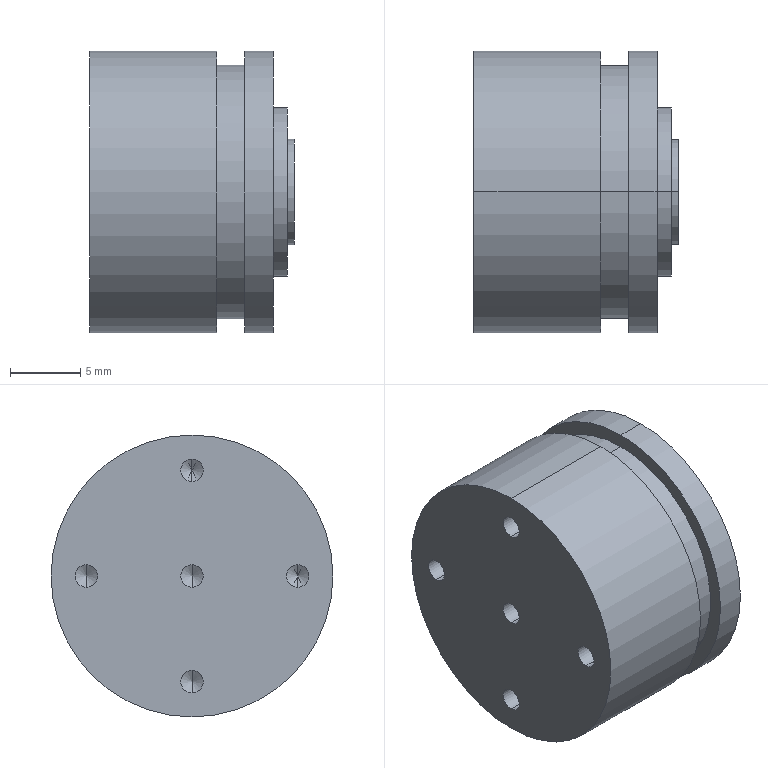Component | SolidWorks | WheelAssembly-1_PressureSensor-1 | 1 solid | 36 faces | box 14.5 x 20 x 20 mm | volume 4051 mm3 | cylinder 20 | cone 10 | plane 6 | commonest cylinder face diameters 1.6 x10 20 x4 7.5 x2 12 x2 18 x2
build123d program:
from build123d import *

# Parameters (mm, degrees)
SKETCH1_R             = 10
BOSS_EXTRUDE1_DEPTH   = 13
CUT_EXTRUDE1_START    = -4
SKETCH2_R             = 10
SKETCH2_R_2           = 9
CUT_EXTRUDE1_DEPTH    = 2
SKETCH3_R             = 6
BOSS_EXTRUDE2_DEPTH   = 1
SKETCH5_R             = 3.75
BOSS_EXTRUDE4_DEPTH   = 0.5
M2_TAPPED_HOLE1_D     = 1.6
M2_TAPPED_HOLE1_DEPTH = 4.7
M2_TAPPED_HOLE1_TIP   = 0.4807


with BuildPart() as part:
    # Sketch1 → Boss-Extrude1 (new body)
    with BuildSketch(Plane.XY):
        with Locations(Location((0, 0, 0), (0, 0, 180))):
            Circle(SKETCH1_R)
    extrude(amount=BOSS_EXTRUDE1_DEPTH)

    # Sketch2 → Cut-Extrude1 (cut)
    with BuildSketch(Plane.XY.offset(13).offset(CUT_EXTRUDE1_START)):
        with Locations(Location((0, 0, 0), (0, 0, 180))):
            Circle(SKETCH2_R)
        Circle(SKETCH2_R_2, mode=Mode.SUBTRACT)
    extrude(amount=CUT_EXTRUDE1_DEPTH, mode=Mode.SUBTRACT)

    # Sketch3 → Boss-Extrude2 (add)
    with BuildSketch(Plane.XY.offset(13)):
        Circle(SKETCH3_R)
    extrude(amount=BOSS_EXTRUDE2_DEPTH)

    # Sketch5 → Boss-Extrude4 (add)
    with BuildSketch(Plane.XY.offset(14)):
        Circle(SKETCH5_R)
    extrude(amount=BOSS_EXTRUDE4_DEPTH)

    # M2 Tapped Hole1
    with Locations(Plane(origin=(0, 0, 0), x_dir=(1, 0, 0), z_dir=(0, 0, -1))):
        with Locations((0, -7.5), (7.5, 0), (0, 7.5), (-7.5, 0), (0, 0)):
            Hole(M2_TAPPED_HOLE1_D / 2, depth=M2_TAPPED_HOLE1_DEPTH)
            with Locations((0, 0, -(M2_TAPPED_HOLE1_DEPTH + M2_TAPPED_HOLE1_TIP / 2))):  # 118° drill point
                Cone(0, M2_TAPPED_HOLE1_D / 2, M2_TAPPED_HOLE1_TIP, mode=Mode.SUBTRACT)


solid = part.part

# Placed as in the assembly
solid = solid.moved(Location((-376, -131.5, -542.97), (0, 90, 0)))
STEP:
#1=COLOUR_RGB('',0.7922,0.8196,0.9333);
#2=FILL_AREA_STYLE_COLOUR('',#1);
#3=FILL_AREA_STYLE('',(#2));
#4=SURFACE_STYLE_FILL_AREA(#3);
#5=SURFACE_SIDE_STYLE('',(#4));
#6=SURFACE_STYLE_USAGE(.BOTH.,#5);
#7=PRESENTATION_STYLE_ASSIGNMENT((#6));
#8=CARTESIAN_POINT('',(-14.618,-5.472,-21.345));
#9=VERTEX_POINT('',#8);
#10=CARTESIAN_POINT('',(-14.618,-5.472,-21.408));
#11=VERTEX_POINT('',#10);
#12=CARTESIAN_POINT('',(-14.618,-5.472,-21.377));
#13=DIRECTION('',(-1.,-0.,0.));
#14=DIRECTION('',(0.,0.,-1.));
#15=AXIS2_PLACEMENT_3D('',#12,#13,#14);
#16=CIRCLE('',#15,0.0315);
#17=EDGE_CURVE('',#9,#11,#16,.T.);
#18=ORIENTED_EDGE('',*,*,#17,.F.);
#19=CARTESIAN_POINT('',(-14.803,-5.472,-21.345));
#20=VERTEX_POINT('',#19);
#21=CARTESIAN_POINT('',(-14.803,-5.472,-21.345));
#22=DIRECTION('',(-1.,-0.,0.));
#23=VECTOR('',#22,39.37);
#24=LINE('',#21,#23);
#25=EDGE_CURVE('',#9,#20,#24,.T.);
#26=ORIENTED_EDGE('',*,*,#25,.T.);
#27=CARTESIAN_POINT('',(-14.803,-5.472,-21.408));
#28=VERTEX_POINT('',#27);
#29=CARTESIAN_POINT('',(-14.803,-5.472,-21.377));
#30=DIRECTION('',(-1.,-0.,0.));
#31=DIRECTION('',(0.,0.,-1.));
#32=AXIS2_PLACEMENT_3D('',#29,#30,#31);
#33=CIRCLE('',#32,0.0315);
#34=EDGE_CURVE('',#20,#28,#33,.T.);
#35=ORIENTED_EDGE('',*,*,#34,.T.);
#36=CARTESIAN_POINT('',(-14.803,-5.472,-21.408));
#37=DIRECTION('',(-1.,-0.,0.));
#38=VECTOR('',#37,39.37);
#39=LINE('',#36,#38);
#40=EDGE_CURVE('',#11,#28,#39,.T.);
#41=ORIENTED_EDGE('',*,*,#40,.F.);
#42=EDGE_LOOP('',(#18,#26,#35,#41));
#43=FACE_OUTER_BOUND('',#42,.T.);
#44=CARTESIAN_POINT('',(-14.803,-5.472,-21.377));
#45=DIRECTION('',(-1.,-0.,0.));
#46=DIRECTION('',(0.,0.,-1.));
#47=AXIS2_PLACEMENT_3D('',#44,#45,#46);
#48=CYLINDRICAL_SURFACE('',#47,0.0315);
#49=ADVANCED_FACE('',(#43),#48,.F.);
#50=CARTESIAN_POINT('',(-14.599,-5.472,-21.377));
#51=VERTEX_POINT('',#50);
#52=CARTESIAN_POINT('',(-14.618,-5.472,-21.408));
#53=DIRECTION('',(-0.515,-0.,-0.8572));
#54=VECTOR('',#53,39.37);
#55=LINE('',#52,#54);
#56=EDGE_CURVE('',#51,#11,#55,.T.);
#57=ORIENTED_EDGE('',*,*,#56,.F.);
#58=CARTESIAN_POINT('',(-14.618,-5.472,-21.345));
#59=DIRECTION('',(-0.515,0.,0.8572));
#60=VECTOR('',#59,39.37);
#61=LINE('',#58,#60);
#62=EDGE_CURVE('',#51,#9,#61,.T.);
#63=ORIENTED_EDGE('',*,*,#62,.T.);
#64=ORIENTED_EDGE('',*,*,#17,.T.);
#65=EDGE_LOOP('',(#57,#63,#64));
#66=FACE_OUTER_BOUND('',#65,.T.);
#67=CARTESIAN_POINT('',(-14.618,-5.472,-21.377));
#68=DIRECTION('',(-1.,-0.,0.));
#69=DIRECTION('',(0.,0.,-1.));
#70=AXIS2_PLACEMENT_3D('',#67,#68,#69);
#71=CONICAL_SURFACE('',#70,0.0315,1.03);
#72=ADVANCED_FACE('',(#66),#71,.F.);
#73=CARTESIAN_POINT('',(-14.618,-5.177,-21.05));
#74=VERTEX_POINT('',#73);
#75=CARTESIAN_POINT('',(-14.618,-5.177,-21.113));
#76=VERTEX_POINT('',#75);
#77=CARTESIAN_POINT('',(-14.618,-5.177,-21.081));
#78=DIRECTION('',(-1.,-0.,0.));
#79=DIRECTION('',(0.,0.,-1.));
#80=AXIS2_PLACEMENT_3D('',#77,#78,#79);
#81=CIRCLE('',#80,0.0315);
#82=EDGE_CURVE('',#74,#76,#81,.T.);
#83=ORIENTED_EDGE('',*,*,#82,.F.);
#84=CARTESIAN_POINT('',(-14.803,-5.177,-21.05));
#85=VERTEX_POINT('',#84);
#86=CARTESIAN_POINT('',(-14.803,-5.177,-21.05));
#87=DIRECTION('',(-1.,-0.,0.));
#88=VECTOR('',#87,39.37);
#89=LINE('',#86,#88);
#90=EDGE_CURVE('',#74,#85,#89,.T.);
#91=ORIENTED_EDGE('',*,*,#90,.T.);
#92=CARTESIAN_POINT('',(-14.803,-5.177,-21.113));
#93=VERTEX_POINT('',#92);
#94=CARTESIAN_POINT('',(-14.803,-5.177,-21.081));
#95=DIRECTION('',(-1.,-0.,0.));
#96=DIRECTION('',(0.,0.,-1.));
#97=AXIS2_PLACEMENT_3D('',#94,#95,#96);
#98=CIRCLE('',#97,0.0315);
#99=EDGE_CURVE('',#85,#93,#98,.T.);
#100=ORIENTED_EDGE('',*,*,#99,.T.);
#101=CARTESIAN_POINT('',(-14.803,-5.177,-21.113));
#102=DIRECTION('',(-1.,-0.,0.));
#103=VECTOR('',#102,39.37);
#104=LINE('',#101,#103);
#105=EDGE_CURVE('',#76,#93,#104,.T.);
#106=ORIENTED_EDGE('',*,*,#105,.F.);
#107=EDGE_LOOP('',(#83,#91,#100,#106));
#108=FACE_OUTER_BOUND('',#107,.T.);
#109=CARTESIAN_POINT('',(-14.803,-5.177,-21.081));
#110=DIRECTION('',(-1.,-0.,0.));
#111=DIRECTION('',(0.,0.,-1.));
#112=AXIS2_PLACEMENT_3D('',#109,#110,#111);
#113=CYLINDRICAL_SURFACE('',#112,0.0315);
#114=ADVANCED_FACE('',(#108),#113,.F.);
#115=CARTESIAN_POINT('',(-14.599,-5.177,-21.081));
#116=VERTEX_POINT('',#115);
#117=CARTESIAN_POINT('',(-14.618,-5.177,-21.113));
#118=DIRECTION('',(-0.515,-0.,-0.8572));
#119=VECTOR('',#118,39.37);
#120=LINE('',#117,#119);
#121=EDGE_CURVE('',#116,#76,#120,.T.);
#122=ORIENTED_EDGE('',*,*,#121,.F.);
#123=CARTESIAN_POINT('',(-14.618,-5.177,-21.05));
#124=DIRECTION('',(-0.515,0.,0.8572));
#125=VECTOR('',#124,39.37);
#126=LINE('',#123,#125);
#127=EDGE_CURVE('',#116,#74,#126,.T.);
#128=ORIENTED_EDGE('',*,*,#127,.T.);
#129=ORIENTED_EDGE('',*,*,#82,.T.);
#130=EDGE_LOOP('',(#122,#128,#129));
#131=FACE_OUTER_BOUND('',#130,.T.);
#132=CARTESIAN_POINT('',(-14.618,-5.177,-21.081));
#133=DIRECTION('',(-1.,-0.,0.));
#134=DIRECTION('',(0.,0.,-1.));
#135=AXIS2_PLACEMENT_3D('',#132,#133,#134);
#136=CONICAL_SURFACE('',#135,0.0315,1.03);
#137=ADVANCED_FACE('',(#131),#136,.F.);
#138=CARTESIAN_POINT('',(-14.618,-4.882,-21.345));
#139=VERTEX_POINT('',#138);
#140=CARTESIAN_POINT('',(-14.618,-4.882,-21.408));
#141=VERTEX_POINT('',#140);
#142=CARTESIAN_POINT('',(-14.618,-4.882,-21.377));
#143=DIRECTION('',(-1.,-0.,0.));
#144=DIRECTION('',(0.,0.,-1.));
#145=AXIS2_PLACEMENT_3D('',#142,#143,#144);
#146=CIRCLE('',#145,0.0315);
#147=EDGE_CURVE('',#139,#141,#146,.T.);
#148=ORIENTED_EDGE('',*,*,#147,.F.);
#149=CARTESIAN_POINT('',(-14.803,-4.882,-21.345));
#150=VERTEX_POINT('',#149);
#151=CARTESIAN_POINT('',(-14.803,-4.882,-21.345));
#152=DIRECTION('',(-1.,-0.,0.));
#153=VECTOR('',#152,39.37);
#154=LINE('',#151,#153);
#155=EDGE_CURVE('',#139,#150,#154,.T.);
#156=ORIENTED_EDGE('',*,*,#155,.T.);
#157=CARTESIAN_POINT('',(-14.803,-4.882,-21.408));
#158=VERTEX_POINT('',#157);
#159=CARTESIAN_POINT('',(-14.803,-4.882,-21.377));
#160=DIRECTION('',(-1.,-0.,0.));
#161=DIRECTION('',(0.,0.,-1.));
#162=AXIS2_PLACEMENT_3D('',#159,#160,#161);
#163=CIRCLE('',#162,0.0315);
#164=EDGE_CURVE('',#150,#158,#163,.T.);
#165=ORIENTED_EDGE('',*,*,#164,.T.);
#166=CARTESIAN_POINT('',(-14.803,-4.882,-21.408));
#167=DIRECTION('',(-1.,-0.,0.));
#168=VECTOR('',#167,39.37);
#169=LINE('',#166,#168);
#170=EDGE_CURVE('',#141,#158,#169,.T.);
#171=ORIENTED_EDGE('',*,*,#170,.F.);
#172=EDGE_LOOP('',(#148,#156,#165,#171));
#173=FACE_OUTER_BOUND('',#172,.T.);
#174=CARTESIAN_POINT('',(-14.803,-4.882,-21.377));
#175=DIRECTION('',(-1.,-0.,0.));
#176=DIRECTION('',(0.,0.,-1.));
#177=AXIS2_PLACEMENT_3D('',#174,#175,#176);
#178=CYLINDRICAL_SURFACE('',#177,0.0315);
#179=ADVANCED_FACE('',(#173),#178,.F.);
#180=CARTESIAN_POINT('',(-14.599,-4.882,-21.377));
#181=VERTEX_POINT('',#180);
#182=CARTESIAN_POINT('',(-14.618,-4.882,-21.408));
#183=DIRECTION('',(-0.515,-0.,-0.8572));
#184=VECTOR('',#183,39.37);
#185=LINE('',#182,#184);
#186=EDGE_CURVE('',#181,#141,#185,.T.);
#187=ORIENTED_EDGE('',*,*,#186,.F.);
#188=CARTESIAN_POINT('',(-14.618,-4.882,-21.345));
#189=DIRECTION('',(-0.515,0.,0.8572));
#190=VECTOR('',#189,39.37);
#191=LINE('',#188,#190);
#192=EDGE_CURVE('',#181,#139,#191,.T.);
#193=ORIENTED_EDGE('',*,*,#192,.T.);
#194=ORIENTED_EDGE('',*,*,#147,.T.);
#195=EDGE_LOOP('',(#187,#193,#194));
#196=FACE_OUTER_BOUND('',#195,.T.);
#197=CARTESIAN_POINT('',(-14.618,-4.882,-21.377));
#198=DIRECTION('',(-1.,-0.,0.));
#199=DIRECTION('',(0.,0.,-1.));
#200=AXIS2_PLACEMENT_3D('',#197,#198,#199);
#201=CONICAL_SURFACE('',#200,0.0315,1.03);
#202=ADVANCED_FACE('',(#196),#201,.F.);
#203=CARTESIAN_POINT('',(-14.618,-5.177,-21.641));
#204=VERTEX_POINT('',#203);
#205=CARTESIAN_POINT('',(-14.618,-5.177,-21.704));
#206=VERTEX_POINT('',#205);
#207=CARTESIAN_POINT('',(-14.618,-5.177,-21.672));
#208=DIRECTION('',(-1.,-0.,0.));
#209=DIRECTION('',(0.,0.,-1.));
#210=AXIS2_PLACEMENT_3D('',#207,#208,#209);
#211=CIRCLE('',#210,0.0315);
#212=EDGE_CURVE('',#204,#206,#211,.T.);
#213=ORIENTED_EDGE('',*,*,#212,.F.);
#214=CARTESIAN_POINT('',(-14.803,-5.177,-21.641));
#215=VERTEX_POINT('',#214);
#216=CARTESIAN_POINT('',(-14.803,-5.177,-21.641));
#217=DIRECTION('',(-1.,-0.,0.));
#218=VECTOR('',#217,39.37);
#219=LINE('',#216,#218);
#220=EDGE_CURVE('',#204,#215,#219,.T.);
#221=ORIENTED_EDGE('',*,*,#220,.T.);
#222=CARTESIAN_POINT('',(-14.803,-5.177,-21.704));
#223=VERTEX_POINT('',#222);
#224=CARTESIAN_POINT('',(-14.803,-5.177,-21.672));
#225=DIRECTION('',(-1.,-0.,0.));
#226=DIRECTION('',(0.,0.,-1.));
#227=AXIS2_PLACEMENT_3D('',#224,#225,#226);
#228=CIRCLE('',#227,0.0315);
#229=EDGE_CURVE('',#215,#223,#228,.T.);
#230=ORIENTED_EDGE('',*,*,#229,.T.);
#231=CARTESIAN_POINT('',(-14.803,-5.177,-21.704));
#232=DIRECTION('',(-1.,-0.,0.));
#233=VECTOR('',#232,39.37);
#234=LINE('',#231,#233);
#235=EDGE_CURVE('',#206,#223,#234,.T.);
#236=ORIENTED_EDGE('',*,*,#235,.F.);
#237=EDGE_LOOP('',(#213,#221,#230,#236));
#238=FACE_OUTER_BOUND('',#237,.T.);
#239=CARTESIAN_POINT('',(-14.803,-5.177,-21.672));
#240=DIRECTION('',(-1.,-0.,0.));
#241=DIRECTION('',(0.,0.,-1.));
#242=AXIS2_PLACEMENT_3D('',#239,#240,#241);
#243=CYLINDRICAL_SURFACE('',#242,0.0315);
#244=ADVANCED_FACE('',(#238),#243,.F.);
#245=CARTESIAN_POINT('',(-14.599,-5.177,-21.672));
#246=VERTEX_POINT('',#245);
#247=CARTESIAN_POINT('',(-14.618,-5.177,-21.704));
#248=DIRECTION('',(-0.515,-0.,-0.8572));
#249=VECTOR('',#248,39.37);
#250=LINE('',#247,#249);
#251=EDGE_CURVE('',#246,#206,#250,.T.);
#252=ORIENTED_EDGE('',*,*,#251,.F.);
#253=CARTESIAN_POINT('',(-14.618,-5.177,-21.641));
#254=DIRECTION('',(-0.515,0.,0.8572));
#255=VECTOR('',#254,39.37);
#256=LINE('',#253,#255);
#257=EDGE_CURVE('',#246,#204,#256,.T.);
#258=ORIENTED_EDGE('',*,*,#257,.T.);
#259=ORIENTED_EDGE('',*,*,#212,.T.);
#260=EDGE_LOOP('',(#252,#258,#259));
#261=FACE_OUTER_BOUND('',#260,.T.);
#262=CARTESIAN_POINT('',(-14.618,-5.177,-21.672));
#263=DIRECTION('',(-1.,-0.,0.));
#264=DIRECTION('',(0.,0.,-1.));
#265=AXIS2_PLACEMENT_3D('',#262,#263,#264);
#266=CONICAL_SURFACE('',#265,0.0315,1.03);
#267=ADVANCED_FACE('',(#261),#266,.F.);
#268=CARTESIAN_POINT('',(-14.618,-5.177,-21.345));
#269=VERTEX_POINT('',#268);
#270=CARTESIAN_POINT('',(-14.618,-5.177,-21.408));
#271=VERTEX_POINT('',#270);
#272=CARTESIAN_POINT('',(-14.618,-5.177,-21.377));
#273=DIRECTION('',(-1.,-0.,0.));
#274=DIRECTION('',(0.,0.,-1.));
#275=AXIS2_PLACEMENT_3D('',#272,#273,#274);
#276=CIRCLE('',#275,0.0315);
#277=EDGE_CURVE('',#269,#271,#276,.T.);
#278=ORIENTED_EDGE('',*,*,#277,.F.);
#279=CARTESIAN_POINT('',(-14.803,-5.177,-21.345));
#280=VERTEX_POINT('',#279);
#281=CARTESIAN_POINT('',(-14.803,-5.177,-21.345));
#282=DIRECTION('',(-1.,-0.,0.));
#283=VECTOR('',#282,39.37);
#284=LINE('',#281,#283);
#285=EDGE_CURVE('',#269,#280,#284,.T.);
#286=ORIENTED_EDGE('',*,*,#285,.T.);
#287=CARTESIAN_POINT('',(-14.803,-5.177,-21.408));
#288=VERTEX_POINT('',#287);
#289=CARTESIAN_POINT('',(-14.803,-5.177,-21.377));
#290=DIRECTION('',(-1.,-0.,0.));
#291=DIRECTION('',(0.,0.,-1.));
#292=AXIS2_PLACEMENT_3D('',#289,#290,#291);
#293=CIRCLE('',#292,0.0315);
#294=EDGE_CURVE('',#280,#288,#293,.T.);
#295=ORIENTED_EDGE('',*,*,#294,.T.);
#296=CARTESIAN_POINT('',(-14.803,-5.177,-21.408));
#297=DIRECTION('',(-1.,-0.,0.));
#298=VECTOR('',#297,39.37);
#299=LINE('',#296,#298);
#300=EDGE_CURVE('',#271,#288,#299,.T.);
#301=ORIENTED_EDGE('',*,*,#300,.F.);
#302=EDGE_LOOP('',(#278,#286,#295,#301));
#303=FACE_OUTER_BOUND('',#302,.T.);
#304=CARTESIAN_POINT('',(-14.803,-5.177,-21.377));
#305=DIRECTION('',(-1.,-0.,0.));
#306=DIRECTION('',(0.,0.,-1.));
#307=AXIS2_PLACEMENT_3D('',#304,#305,#306);
#308=CYLINDRICAL_SURFACE('',#307,0.0315);
#309=ADVANCED_FACE('',(#303),#308,.F.);
#310=CARTESIAN_POINT('',(-14.599,-5.177,-21.377));
#311=VERTEX_POINT('',#310);
#312=CARTESIAN_POINT('',(-14.618,-5.177,-21.408));
#313=DIRECTION('',(-0.515,-0.,-0.8572));
#314=VECTOR('',#313,39.37);
#315=LINE('',#312,#314);
#316=EDGE_CURVE('',#311,#271,#315,.T.);
#317=ORIENTED_EDGE('',*,*,#316,.F.);
#318=CARTESIAN_POINT('',(-14.618,-5.177,-21.345));
#319=DIRECTION('',(-0.515,0.,0.8572));
#320=VECTOR('',#319,39.37);
#321=LINE('',#318,#320);
#322=EDGE_CURVE('',#311,#269,#321,.T.);
#323=ORIENTED_EDGE('',*,*,#322,.T.);
#324=ORIENTED_EDGE('',*,*,#277,.T.);
#325=EDGE_LOOP('',(#317,#323,#324));
#326=FACE_OUTER_BOUND('',#325,.T.);
#327=CARTESIAN_POINT('',(-14.618,-5.177,-21.377));
#328=DIRECTION('',(-1.,-0.,0.));
#329=DIRECTION('',(0.,0.,-1.));
#330=AXIS2_PLACEMENT_3D('',#327,#328,#329);
#331=CONICAL_SURFACE('',#330,0.0315,1.03);
#332=ADVANCED_FACE('',(#326),#331,.F.);
#333=CARTESIAN_POINT('',(-14.232,-5.177,-21.229));
#334=VERTEX_POINT('',#333);
#335=CARTESIAN_POINT('',(-14.232,-5.177,-21.524));
#336=VERTEX_POINT('',#335);
#337=CARTESIAN_POINT('',(-14.232,-5.177,-21.377));
#338=DIRECTION('',(1.,0.,-0.));
#339=DIRECTION('',(0.,0.,1.));
#340=AXIS2_PLACEMENT_3D('',#337,#338,#339);
#341=CIRCLE('',#340,0.1476);
#342=EDGE_CURVE('',#334,#336,#341,.T.);
#343=ORIENTED_EDGE('',*,*,#342,.F.);
#344=CARTESIAN_POINT('',(-14.252,-5.177,-21.229));
#345=VERTEX_POINT('',#344);
#346=CARTESIAN_POINT('',(-14.232,-5.177,-21.229));
#347=DIRECTION('',(-1.,-0.,0.));
#348=VECTOR('',#347,39.37);
#349=LINE('',#346,#348);
#350=EDGE_CURVE('',#334,#345,#349,.T.);
#351=ORIENTED_EDGE('',*,*,#350,.T.);
#352=CARTESIAN_POINT('',(-14.252,-5.177,-21.524));
#353=VERTEX_POINT('',#352);
#354=CARTESIAN_POINT('',(-14.252,-5.177,-21.377));
#355=DIRECTION('',(1.,0.,-0.));
#356=DIRECTION('',(0.,0.,1.));
#357=AXIS2_PLACEMENT_3D('',#354,#355,#356);
#358=CIRCLE('',#357,0.1476);
#359=EDGE_CURVE('',#345,#353,#358,.T.);
#360=ORIENTED_EDGE('',*,*,#359,.T.);
#361=CARTESIAN_POINT('',(-14.232,-5.177,-21.524));
#362=DIRECTION('',(-1.,-0.,0.));
#363=VECTOR('',#362,39.37);
#364=LINE('',#361,#363);
#365=EDGE_CURVE('',#336,#353,#364,.T.);
#366=ORIENTED_EDGE('',*,*,#365,.F.);
#367=EDGE_LOOP('',(#343,#351,#360,#366));
#368=FACE_OUTER_BOUND('',#367,.T.);
#369=CARTESIAN_POINT('',(-14.232,-5.177,-21.377));
#370=DIRECTION('',(-1.,-0.,0.));
#371=DIRECTION('',(0.,-0.,-1.));
#372=AXIS2_PLACEMENT_3D('',#369,#370,#371);
#373=CYLINDRICAL_SURFACE('',#372,0.1476);
#374=ADVANCED_FACE('',(#368),#373,.T.);
#375=CARTESIAN_POINT('',(-14.252,-5.177,-21.141));
#376=VERTEX_POINT('',#375);
#377=CARTESIAN_POINT('',(-14.252,-5.177,-21.613));
#378=VERTEX_POINT('',#377);
#379=CARTESIAN_POINT('',(-14.252,-5.177,-21.377));
#380=DIRECTION('',(1.,0.,-0.));
#381=DIRECTION('',(0.,0.,1.));
#382=AXIS2_PLACEMENT_3D('',#379,#380,#381);
#383=CIRCLE('',#382,0.2362);
#384=EDGE_CURVE('',#376,#378,#383,.T.);
#385=ORIENTED_EDGE('',*,*,#384,.F.);
#386=CARTESIAN_POINT('',(-14.291,-5.177,-21.141));
#387=VERTEX_POINT('',#386);
#388=CARTESIAN_POINT('',(-14.252,-5.177,-21.141));
#389=DIRECTION('',(-1.,-0.,0.));
#390=VECTOR('',#389,39.37);
#391=LINE('',#388,#390);
#392=EDGE_CURVE('',#376,#387,#391,.T.);
#393=ORIENTED_EDGE('',*,*,#392,.T.);
#394=CARTESIAN_POINT('',(-14.291,-5.177,-21.613));
#395=VERTEX_POINT('',#394);
#396=CARTESIAN_POINT('',(-14.291,-5.177,-21.377));
#397=DIRECTION('',(1.,0.,-0.));
#398=DIRECTION('',(0.,0.,1.));
#399=AXIS2_PLACEMENT_3D('',#396,#397,#398);
#400=CIRCLE('',#399,0.2362);
#401=EDGE_CURVE('',#387,#395,#400,.T.);
#402=ORIENTED_EDGE('',*,*,#401,.T.);
#403=CARTESIAN_POINT('',(-14.252,-5.177,-21.613));
#404=DIRECTION('',(-1.,-0.,0.));
#405=VECTOR('',#404,39.37);
#406=LINE('',#403,#405);
#407=EDGE_CURVE('',#378,#395,#406,.T.);
#408=ORIENTED_EDGE('',*,*,#407,.F.);
#409=EDGE_LOOP('',(#385,#393,#402,#408));
#410=FACE_OUTER_BOUND('',#409,.T.);
#411=CARTESIAN_POINT('',(-14.252,-5.177,-21.377));
#412=DIRECTION('',(-1.,-0.,0.));
#413=DIRECTION('',(0.,-0.,-1.));
#414=AXIS2_PLACEMENT_3D('',#411,#412,#413);
#415=CYLINDRICAL_SURFACE('',#414,0.2362);
#416=ADVANCED_FACE('',(#410),#415,.T.);
#417=CARTESIAN_POINT('',(-14.291,-5.177,-20.983));
#418=VERTEX_POINT('',#417);
#419=CARTESIAN_POINT('',(-14.291,-5.177,-21.77));
#420=VERTEX_POINT('',#419);
#421=CARTESIAN_POINT('',(-14.291,-5.177,-21.377));
#422=DIRECTION('',(1.,0.,-0.));
#423=DIRECTION('',(0.,0.,1.));
#424=AXIS2_PLACEMENT_3D('',#421,#422,#423);
#425=CIRCLE('',#424,0.3937);
#426=EDGE_CURVE('',#418,#420,#425,.T.);
#427=ORIENTED_EDGE('',*,*,#426,.F.);
#428=CARTESIAN_POINT('',(-14.37,-5.177,-20.983));
#429=VERTEX_POINT('',#428);
#430=CARTESIAN_POINT('',(-14.291,-5.177,-20.983));
#431=DIRECTION('',(-1.,-0.,0.));
#432=VECTOR('',#431,39.37);
#433=LINE('',#430,#432);
#434=EDGE_CURVE('',#418,#429,#433,.T.);
#435=ORIENTED_EDGE('',*,*,#434,.T.);
#436=CARTESIAN_POINT('',(-14.37,-5.177,-21.77));
#437=VERTEX_POINT('',#436);
#438=CARTESIAN_POINT('',(-14.37,-5.177,-21.377));
#439=DIRECTION('',(1.,0.,-0.));
#440=DIRECTION('',(0.,0.,1.));
#441=AXIS2_PLACEMENT_3D('',#438,#439,#440);
#442=CIRCLE('',#441,0.3937);
#443=EDGE_CURVE('',#429,#437,#442,.T.);
#444=ORIENTED_EDGE('',*,*,#443,.T.);
#445=CARTESIAN_POINT('',(-14.291,-5.177,-21.77));
#446=DIRECTION('',(-1.,-0.,0.));
#447=VECTOR('',#446,39.37);
#448=LINE('',#445,#447);
#449=EDGE_CURVE('',#420,#437,#448,.T.);
#450=ORIENTED_EDGE('',*,*,#449,.F.);
#451=EDGE_LOOP('',(#427,#435,#444,#450));
#452=FACE_OUTER_BOUND('',#451,.T.);
#453=CARTESIAN_POINT('',(-14.291,-5.177,-21.377));
#454=DIRECTION('',(-1.,-0.,0.));
#455=DIRECTION('',(0.,-0.,-1.));
#456=AXIS2_PLACEMENT_3D('',#453,#454,#455);
#457=CYLINDRICAL_SURFACE('',#456,0.3937);
#458=ADVANCED_FACE('',(#452),#457,.T.);
#459=CARTESIAN_POINT('',(-14.449,-5.177,-21.022));
#460=VERTEX_POINT('',#459);
#461=CARTESIAN_POINT('',(-14.449,-5.177,-21.731));
#462=VERTEX_POINT('',#461);
#463=CARTESIAN_POINT('',(-14.449,-5.177,-21.377));
#464=DIRECTION('',(1.,0.,-0.));
#465=DIRECTION('',(0.,0.,1.));
#466=AXIS2_PLACEMENT_3D('',#463,#464,#465);
#467=CIRCLE('',#466,0.3543);
#468=EDGE_CURVE('',#460,#462,#467,.T.);
#469=ORIENTED_EDGE('',*,*,#468,.T.);
#470=CARTESIAN_POINT('',(-14.37,-5.177,-21.731));
#471=VERTEX_POINT('',#470);
#472=CARTESIAN_POINT('',(-14.449,-5.177,-21.731));
#473=DIRECTION('',(1.,0.,-0.));
#474=VECTOR('',#473,39.37);
#475=LINE('',#472,#474);
#476=EDGE_CURVE('',#462,#471,#475,.T.);
#477=ORIENTED_EDGE('',*,*,#476,.T.);
#478=CARTESIAN_POINT('',(-14.37,-5.177,-21.022));
#479=VERTEX_POINT('',#478);
#480=CARTESIAN_POINT('',(-14.37,-5.177,-21.377));
#481=DIRECTION('',(1.,0.,-0.));
#482=DIRECTION('',(0.,0.,1.));
#483=AXIS2_PLACEMENT_3D('',#480,#481,#482);
#484=CIRCLE('',#483,0.3543);
#485=EDGE_CURVE('',#479,#471,#484,.T.);
#486=ORIENTED_EDGE('',*,*,#485,.F.);
#487=CARTESIAN_POINT('',(-14.449,-5.177,-21.022));
#488=DIRECTION('',(1.,0.,-0.));
#489=VECTOR('',#488,39.37);
#490=LINE('',#487,#489);
#491=EDGE_CURVE('',#460,#479,#490,.T.);
#492=ORIENTED_EDGE('',*,*,#491,.F.);
#493=EDGE_LOOP('',(#469,#477,#486,#492));
#494=FACE_OUTER_BOUND('',#493,.T.);
#495=CARTESIAN_POINT('',(-14.449,-5.177,-21.377));
#496=DIRECTION('',(1.,0.,-0.));
#497=DIRECTION('',(0.,0.,1.));
#498=AXIS2_PLACEMENT_3D('',#495,#496,#497);
#499=CYLINDRICAL_SURFACE('',#498,0.3543);
#500=ADVANCED_FACE('',(#494),#499,.T.);
#501=CARTESIAN_POINT('',(-14.449,-5.177,-20.983));
#502=VERTEX_POINT('',#501);
#503=CARTESIAN_POINT('',(-14.449,-5.177,-21.77));
#504=VERTEX_POINT('',#503);
#505=CARTESIAN_POINT('',(-14.449,-5.177,-21.377));
#506=DIRECTION('',(1.,0.,-0.));
#507=DIRECTION('',(0.,0.,1.));
#508=AXIS2_PLACEMENT_3D('',#505,#506,#507);
#509=CIRCLE('',#508,0.3937);
#510=EDGE_CURVE('',#502,#504,#509,.T.);
#511=ORIENTED_EDGE('',*,*,#510,.F.);
#512=CARTESIAN_POINT('',(-14.803,-5.177,-20.983));
#513=VERTEX_POINT('',#512);
#514=CARTESIAN_POINT('',(-14.291,-5.177,-20.983));
#515=DIRECTION('',(-1.,-0.,0.));
#516=VECTOR('',#515,39.37);
#517=LINE('',#514,#516);
#518=EDGE_CURVE('',#502,#513,#517,.T.);
#519=ORIENTED_EDGE('',*,*,#518,.T.);
#520=CARTESIAN_POINT('',(-14.803,-5.177,-21.77));
#521=VERTEX_POINT('',#520);
#522=CARTESIAN_POINT('',(-14.803,-5.177,-21.377));
#523=DIRECTION('',(1.,0.,-0.));
#524=DIRECTION('',(0.,0.,1.));
#525=AXIS2_PLACEMENT_3D('',#522,#523,#524);
#526=CIRCLE('',#525,0.3937);
#527=EDGE_CURVE('',#513,#521,#526,.T.);
#528=ORIENTED_EDGE('',*,*,#527,.T.);
#529=CARTESIAN_POINT('',(-14.291,-5.177,-21.77));
#530=DIRECTION('',(-1.,-0.,0.));
#531=VECTOR('',#530,39.37);
#532=LINE('',#529,#531);
#533=EDGE_CURVE('',#504,#521,#532,.T.);
#534=ORIENTED_EDGE('',*,*,#533,.F.);
#535=EDGE_LOOP('',(#511,#519,#528,#534));
#536=FACE_OUTER_BOUND('',#535,.T.);
#537=CARTESIAN_POINT('',(-14.291,-5.177,-21.377));
#538=DIRECTION('',(-1.,-0.,0.));
#539=DIRECTION('',(0.,-0.,-1.));
#540=AXIS2_PLACEMENT_3D('',#537,#538,#539);
#541=CYLINDRICAL_SURFACE('',#540,0.3937);
#542=ADVANCED_FACE('',(#536),#541,.T.);
#543=CARTESIAN_POINT('',(-14.803,-5.472,-21.377));
#544=DIRECTION('',(-1.,-0.,0.));
#545=DIRECTION('',(0.,0.,-1.));
#546=AXIS2_PLACEMENT_3D('',#543,#544,#545);
#547=CIRCLE('',#546,0.0315);
#548=EDGE_CURVE('',#28,#20,#547,.T.);
#549=ORIENTED_EDGE('',*,*,#548,.F.);
#550=ORIENTED_EDGE('',*,*,#34,.F.);
#551=EDGE_LOOP('',(#549,#550));
#552=FACE_BOUND('',#551,.T.);
#553=CARTESIAN_POINT('',(-14.803,-5.177,-21.672));
#554=DIRECTION('',(-1.,-0.,0.));
#555=DIRECTION('',(0.,0.,-1.));
#556=AXIS2_PLACEMENT_3D('',#553,#554,#555);
#557=CIRCLE('',#556,0.0315);
#558=EDGE_CURVE('',#223,#215,#557,.T.);
#559=ORIENTED_EDGE('',*,*,#558,.F.);
#560=ORIENTED_EDGE('',*,*,#229,.F.);
#561=EDGE_LOOP('',(#559,#560));
#562=FACE_BOUND('',#561,.T.);
#563=CARTESIAN_POINT('',(-14.803,-5.177,-21.377));
#564=DIRECTION('',(-1.,-0.,0.));
#565=DIRECTION('',(0.,0.,-1.));
#566=AXIS2_PLACEMENT_3D('',#563,#564,#565);
#567=CIRCLE('',#566,0.0315);
#568=EDGE_CURVE('',#288,#280,#567,.T.);
#569=ORIENTED_EDGE('',*,*,#568,.F.);
#570=ORIENTED_EDGE('',*,*,#294,.F.);
#571=EDGE_LOOP('',(#569,#570));
#572=FACE_BOUND('',#571,.T.);
#573=CARTESIAN_POINT('',(-14.803,-5.177,-21.377));
#574=DIRECTION('',(1.,0.,-0.));
#575=DIRECTION('',(0.,0.,1.));
#576=AXIS2_PLACEMENT_3D('',#573,#574,#575);
#577=CIRCLE('',#576,0.3937);
#578=EDGE_CURVE('',#521,#513,#577,.T.);
#579=ORIENTED_EDGE('',*,*,#578,.F.);
#580=ORIENTED_EDGE('',*,*,#527,.F.);
#581=EDGE_LOOP('',(#579,#580));
#582=FACE_OUTER_BOUND('',#581,.T.);
#583=CARTESIAN_POINT('',(-14.803,-4.882,-21.377));
#584=DIRECTION('',(-1.,-0.,0.));
#585=DIRECTION('',(0.,0.,-1.));
#586=AXIS2_PLACEMENT_3D('',#583,#584,#585);
#587=CIRCLE('',#586,0.0315);
#588=EDGE_CURVE('',#158,#150,#587,.T.);
#589=ORIENTED_EDGE('',*,*,#588,.F.);
#590=ORIENTED_EDGE('',*,*,#164,.F.);
#591=EDGE_LOOP('',(#589,#590));
#592=FACE_BOUND('',#591,.T.);
#593=CARTESIAN_POINT('',(-14.803,-5.177,-21.081));
#594=DIRECTION('',(-1.,-0.,0.));
#595=DIRECTION('',(0.,0.,-1.));
#596=AXIS2_PLACEMENT_3D('',#593,#594,#595);
#597=CIRCLE('',#596,0.0315);
#598=EDGE_CURVE('',#93,#85,#597,.T.);
#599=ORIENTED_EDGE('',*,*,#598,.F.);
#600=ORIENTED_EDGE('',*,*,#99,.F.);
#601=EDGE_LOOP('',(#599,#600));
#602=FACE_BOUND('',#601,.T.);
#603=CARTESIAN_POINT('',(-14.803,-5.177,-21.377));
#604=DIRECTION('',(1.,0.,-0.));
#605=DIRECTION('',(0.,0.,1.));
#606=AXIS2_PLACEMENT_3D('',#603,#604,#605);
#607=PLANE('',#606);
#608=ADVANCED_FACE('',(#552,#562,#572,#582,#592,#602),#607,.F.);
#609=ORIENTED_EDGE('',*,*,#518,.F.);
#610=CARTESIAN_POINT('',(-14.449,-5.177,-21.377));
#611=DIRECTION('',(1.,0.,-0.));
#612=DIRECTION('',(0.,0.,1.));
#613=AXIS2_PLACEMENT_3D('',#610,#611,#612);
#614=CIRCLE('',#613,0.3937);
#615=EDGE_CURVE('',#504,#502,#614,.T.);
#616=ORIENTED_EDGE('',*,*,#615,.F.);
#617=ORIENTED_EDGE('',*,*,#533,.T.);
#618=ORIENTED_EDGE('',*,*,#578,.T.);
#619=EDGE_LOOP('',(#609,#616,#617,#618));
#620=FACE_OUTER_BOUND('',#619,.T.);
#621=CARTESIAN_POINT('',(-14.291,-5.177,-21.377));
#622=DIRECTION('',(-1.,-0.,0.));
#623=DIRECTION('',(0.,-0.,-1.));
#624=AXIS2_PLACEMENT_3D('',#621,#622,#623);
#625=CYLINDRICAL_SURFACE('',#624,0.3937);
#626=ADVANCED_FACE('',(#620),#625,.T.);
#627=ORIENTED_EDGE('',*,*,#468,.F.);
#628=CARTESIAN_POINT('',(-14.449,-5.177,-21.377));
#629=DIRECTION('',(1.,0.,-0.));
#630=DIRECTION('',(0.,0.,1.));
#631=AXIS2_PLACEMENT_3D('',#628,#629,#630);
#632=CIRCLE('',#631,0.3543);
#633=EDGE_CURVE('',#462,#460,#632,.T.);
#634=ORIENTED_EDGE('',*,*,#633,.F.);
#635=EDGE_LOOP('',(#627,#634));
#636=FACE_BOUND('',#635,.T.);
#637=ORIENTED_EDGE('',*,*,#615,.T.);
#638=ORIENTED_EDGE('',*,*,#510,.T.);
#639=EDGE_LOOP('',(#637,#638));
#640=FACE_OUTER_BOUND('',#639,.T.);
#641=CARTESIAN_POINT('',(-14.449,-5.177,-21.377));
#642=DIRECTION('',(1.,0.,-0.));
#643=DIRECTION('',(0.,0.,1.));
#644=AXIS2_PLACEMENT_3D('',#641,#642,#643);
#645=PLANE('',#644);
#646=ADVANCED_FACE('',(#636,#640),#645,.T.);
#647=ORIENTED_EDGE('',*,*,#485,.T.);
#648=CARTESIAN_POINT('',(-14.37,-5.177,-21.377));
#649=DIRECTION('',(1.,0.,-0.));
#650=DIRECTION('',(0.,0.,1.));
#651=AXIS2_PLACEMENT_3D('',#648,#649,#650);
#652=CIRCLE('',#651,0.3543);
#653=EDGE_CURVE('',#471,#479,#652,.T.);
#654=ORIENTED_EDGE('',*,*,#653,.T.);
#655=EDGE_LOOP('',(#647,#654));
#656=FACE_BOUND('',#655,.T.);
#657=CARTESIAN_POINT('',(-14.37,-5.177,-21.377));
#658=DIRECTION('',(1.,0.,-0.));
#659=DIRECTION('',(0.,0.,1.));
#660=AXIS2_PLACEMENT_3D('',#657,#658,#659);
#661=CIRCLE('',#660,0.3937);
#662=EDGE_CURVE('',#437,#429,#661,.T.);
#663=ORIENTED_EDGE('',*,*,#662,.F.);
#664=ORIENTED_EDGE('',*,*,#443,.F.);
#665=EDGE_LOOP('',(#663,#664));
#666=FACE_OUTER_BOUND('',#665,.T.);
#667=CARTESIAN_POINT('',(-14.37,-5.177,-21.377));
#668=DIRECTION('',(1.,0.,-0.));
#669=DIRECTION('',(0.,0.,1.));
#670=AXIS2_PLACEMENT_3D('',#667,#668,#669);
#671=PLANE('',#670);
#672=ADVANCED_FACE('',(#656,#666),#671,.F.);
#673=ORIENTED_EDGE('',*,*,#476,.F.);
#674=ORIENTED_EDGE('',*,*,#633,.T.);
#675=ORIENTED_EDGE('',*,*,#491,.T.);
#676=ORIENTED_EDGE('',*,*,#653,.F.);
#677=EDGE_LOOP('',(#673,#674,#675,#676));
#678=FACE_OUTER_BOUND('',#677,.T.);
#679=CARTESIAN_POINT('',(-14.449,-5.177,-21.377));
#680=DIRECTION('',(1.,0.,-0.));
#681=DIRECTION('',(0.,0.,1.));
#682=AXIS2_PLACEMENT_3D('',#679,#680,#681);
#683=CYLINDRICAL_SURFACE('',#682,0.3543);
#684=ADVANCED_FACE('',(#678),#683,.T.);
#685=CARTESIAN_POINT('',(-14.291,-5.177,-21.377));
#686=DIRECTION('',(1.,0.,-0.));
#687=DIRECTION('',(0.,0.,1.));
#688=AXIS2_PLACEMENT_3D('',#685,#686,#687);
#689=CIRCLE('',#688,0.2362);
#690=EDGE_CURVE('',#395,#387,#689,.T.);
#691=ORIENTED_EDGE('',*,*,#690,.F.);
#692=ORIENTED_EDGE('',*,*,#401,.F.);
#693=EDGE_LOOP('',(#691,#692));
#694=FACE_BOUND('',#693,.T.);
#695=CARTESIAN_POINT('',(-14.291,-5.177,-21.377));
#696=DIRECTION('',(1.,0.,-0.));
#697=DIRECTION('',(0.,0.,1.));
#698=AXIS2_PLACEMENT_3D('',#695,#696,#697);
#699=CIRCLE('',#698,0.3937);
#700=EDGE_CURVE('',#420,#418,#699,.T.);
#701=ORIENTED_EDGE('',*,*,#700,.T.);
#702=ORIENTED_EDGE('',*,*,#426,.T.);
#703=EDGE_LOOP('',(#701,#702));
#704=FACE_OUTER_BOUND('',#703,.T.);
#705=CARTESIAN_POINT('',(-14.291,-5.177,-21.377));
#706=DIRECTION('',(1.,0.,-0.));
#707=DIRECTION('',(0.,0.,1.));
#708=AXIS2_PLACEMENT_3D('',#705,#706,#707);
#709=PLANE('',#708);
#710=ADVANCED_FACE('',(#694,#704),#709,.T.);
#711=ORIENTED_EDGE('',*,*,#434,.F.);
#712=ORIENTED_EDGE('',*,*,#700,.F.);
#713=ORIENTED_EDGE('',*,*,#449,.T.);
#714=ORIENTED_EDGE('',*,*,#662,.T.);
#715=EDGE_LOOP('',(#711,#712,#713,#714));
#716=FACE_OUTER_BOUND('',#715,.T.);
#717=CARTESIAN_POINT('',(-14.291,-5.177,-21.377));
#718=DIRECTION('',(-1.,-0.,0.));
#719=DIRECTION('',(0.,-0.,-1.));
#720=AXIS2_PLACEMENT_3D('',#717,#718,#719);
#721=CYLINDRICAL_SURFACE('',#720,0.3937);
#722=ADVANCED_FACE('',(#716),#721,.T.);
#723=ORIENTED_EDGE('',*,*,#392,.F.);
#724=CARTESIAN_POINT('',(-14.252,-5.177,-21.377));
#725=DIRECTION('',(1.,0.,-0.));
#726=DIRECTION('',(0.,0.,1.));
#727=AXIS2_PLACEMENT_3D('',#724,#725,#726);
#728=CIRCLE('',#727,0.2362);
#729=EDGE_CURVE('',#378,#376,#728,.T.);
#730=ORIENTED_EDGE('',*,*,#729,.F.);
#731=ORIENTED_EDGE('',*,*,#407,.T.);
#732=ORIENTED_EDGE('',*,*,#690,.T.);
#733=EDGE_LOOP('',(#723,#730,#731,#732));
#734=FACE_OUTER_BOUND('',#733,.T.);
#735=CARTESIAN_POINT('',(-14.252,-5.177,-21.377));
#736=DIRECTION('',(-1.,-0.,0.));
#737=DIRECTION('',(0.,-0.,-1.));
#738=AXIS2_PLACEMENT_3D('',#735,#736,#737);
#739=CYLINDRICAL_SURFACE('',#738,0.2362);
#740=ADVANCED_FACE('',(#734),#739,.T.);
#741=CARTESIAN_POINT('',(-14.252,-5.177,-21.377));
#742=DIRECTION('',(1.,0.,-0.));
#743=DIRECTION('',(0.,0.,1.));
#744=AXIS2_PLACEMENT_3D('',#741,#742,#743);
#745=CIRCLE('',#744,0.1476);
#746=EDGE_CURVE('',#353,#345,#745,.T.);
#747=ORIENTED_EDGE('',*,*,#746,.F.);
#748=ORIENTED_EDGE('',*,*,#359,.F.);
#749=EDGE_LOOP('',(#747,#748));
#750=FACE_BOUND('',#749,.T.);
#751=ORIENTED_EDGE('',*,*,#729,.T.);
#752=ORIENTED_EDGE('',*,*,#384,.T.);
#753=EDGE_LOOP('',(#751,#752));
#754=FACE_OUTER_BOUND('',#753,.T.);
#755=CARTESIAN_POINT('',(-14.252,-5.177,-21.377));
#756=DIRECTION('',(1.,0.,-0.));
#757=DIRECTION('',(0.,0.,1.));
#758=AXIS2_PLACEMENT_3D('',#755,#756,#757);
#759=PLANE('',#758);
#760=ADVANCED_FACE('',(#750,#754),#759,.T.);
#761=ORIENTED_EDGE('',*,*,#350,.F.);
#762=CARTESIAN_POINT('',(-14.232,-5.177,-21.377));
#763=DIRECTION('',(1.,0.,-0.));
#764=DIRECTION('',(0.,0.,1.));
#765=AXIS2_PLACEMENT_3D('',#762,#763,#764);
#766=CIRCLE('',#765,0.1476);
#767=EDGE_CURVE('',#336,#334,#766,.T.);
#768=ORIENTED_EDGE('',*,*,#767,.F.);
#769=ORIENTED_EDGE('',*,*,#365,.T.);
#770=ORIENTED_EDGE('',*,*,#746,.T.);
#771=EDGE_LOOP('',(#761,#768,#769,#770));
#772=FACE_OUTER_BOUND('',#771,.T.);
#773=CARTESIAN_POINT('',(-14.232,-5.177,-21.377));
#774=DIRECTION('',(-1.,-0.,0.));
#775=DIRECTION('',(0.,-0.,-1.));
#776=AXIS2_PLACEMENT_3D('',#773,#774,#775);
#777=CYLINDRICAL_SURFACE('',#776,0.1476);
#778=ADVANCED_FACE('',(#772),#777,.T.);
#779=ORIENTED_EDGE('',*,*,#767,.T.);
#780=ORIENTED_EDGE('',*,*,#342,.T.);
#781=EDGE_LOOP('',(#779,#780));
#782=FACE_OUTER_BOUND('',#781,.T.);
#783=CARTESIAN_POINT('',(-14.232,-5.177,-21.377));
#784=DIRECTION('',(1.,0.,-0.));
#785=DIRECTION('',(0.,0.,1.));
#786=AXIS2_PLACEMENT_3D('',#783,#784,#785);
#787=PLANE('',#786);
#788=ADVANCED_FACE('',(#782),#787,.T.);
#789=ORIENTED_EDGE('',*,*,#322,.F.);
#790=ORIENTED_EDGE('',*,*,#316,.T.);
#791=CARTESIAN_POINT('',(-14.618,-5.177,-21.377));
#792=DIRECTION('',(-1.,-0.,0.));
#793=DIRECTION('',(0.,0.,-1.));
#794=AXIS2_PLACEMENT_3D('',#791,#792,#793);
#795=CIRCLE('',#794,0.0315);
#796=EDGE_CURVE('',#271,#269,#795,.T.);
#797=ORIENTED_EDGE('',*,*,#796,.T.);
#798=EDGE_LOOP('',(#789,#790,#797));
#799=FACE_OUTER_BOUND('',#798,.T.);
#800=CARTESIAN_POINT('',(-14.618,-5.177,-21.377));
#801=DIRECTION('',(-1.,-0.,0.));
#802=DIRECTION('',(0.,0.,-1.));
#803=AXIS2_PLACEMENT_3D('',#800,#801,#802);
#804=CONICAL_SURFACE('',#803,0.0315,1.03);
#805=ADVANCED_FACE('',(#799),#804,.F.);
#806=ORIENTED_EDGE('',*,*,#285,.F.);
#807=ORIENTED_EDGE('',*,*,#796,.F.);
#808=ORIENTED_EDGE('',*,*,#300,.T.);
#809=ORIENTED_EDGE('',*,*,#568,.T.);
#810=EDGE_LOOP('',(#806,#807,#808,#809));
#811=FACE_OUTER_BOUND('',#810,.T.);
#812=CARTESIAN_POINT('',(-14.803,-5.177,-21.377));
#813=DIRECTION('',(-1.,-0.,0.));
#814=DIRECTION('',(0.,0.,-1.));
#815=AXIS2_PLACEMENT_3D('',#812,#813,#814);
#816=CYLINDRICAL_SURFACE('',#815,0.0315);
#817=ADVANCED_FACE('',(#811),#816,.F.);
#818=ORIENTED_EDGE('',*,*,#257,.F.);
#819=ORIENTED_EDGE('',*,*,#251,.T.);
#820=CARTESIAN_POINT('',(-14.618,-5.177,-21.672));
#821=DIRECTION('',(-1.,-0.,0.));
#822=DIRECTION('',(0.,0.,-1.));
#823=AXIS2_PLACEMENT_3D('',#820,#821,#822);
#824=CIRCLE('',#823,0.0315);
#825=EDGE_CURVE('',#206,#204,#824,.T.);
#826=ORIENTED_EDGE('',*,*,#825,.T.);
#827=EDGE_LOOP('',(#818,#819,#826));
#828=FACE_OUTER_BOUND('',#827,.T.);
#829=CARTESIAN_POINT('',(-14.618,-5.177,-21.672));
#830=DIRECTION('',(-1.,-0.,0.));
#831=DIRECTION('',(0.,0.,-1.));
#832=AXIS2_PLACEMENT_3D('',#829,#830,#831);
#833=CONICAL_SURFACE('',#832,0.0315,1.03);
#834=ADVANCED_FACE('',(#828),#833,.F.);
#835=ORIENTED_EDGE('',*,*,#220,.F.);
#836=ORIENTED_EDGE('',*,*,#825,.F.);
#837=ORIENTED_EDGE('',*,*,#235,.T.);
#838=ORIENTED_EDGE('',*,*,#558,.T.);
#839=EDGE_LOOP('',(#835,#836,#837,#838));
#840=FACE_OUTER_BOUND('',#839,.T.);
#841=CARTESIAN_POINT('',(-14.803,-5.177,-21.672));
#842=DIRECTION('',(-1.,-0.,0.));
#843=DIRECTION('',(0.,0.,-1.));
#844=AXIS2_PLACEMENT_3D('',#841,#842,#843);
#845=CYLINDRICAL_SURFACE('',#844,0.0315);
#846=ADVANCED_FACE('',(#840),#845,.F.);
#847=ORIENTED_EDGE('',*,*,#192,.F.);
#848=ORIENTED_EDGE('',*,*,#186,.T.);
#849=CARTESIAN_POINT('',(-14.618,-4.882,-21.377));
#850=DIRECTION('',(-1.,-0.,0.));
#851=DIRECTION('',(0.,0.,-1.));
#852=AXIS2_PLACEMENT_3D('',#849,#850,#851);
#853=CIRCLE('',#852,0.0315);
#854=EDGE_CURVE('',#141,#139,#853,.T.);
#855=ORIENTED_EDGE('',*,*,#854,.T.);
#856=EDGE_LOOP('',(#847,#848,#855));
#857=FACE_OUTER_BOUND('',#856,.T.);
#858=CARTESIAN_POINT('',(-14.618,-4.882,-21.377));
#859=DIRECTION('',(-1.,-0.,0.));
#860=DIRECTION('',(0.,0.,-1.));
#861=AXIS2_PLACEMENT_3D('',#858,#859,#860);
#862=CONICAL_SURFACE('',#861,0.0315,1.03);
#863=ADVANCED_FACE('',(#857),#862,.F.);
#864=ORIENTED_EDGE('',*,*,#155,.F.);
#865=ORIENTED_EDGE('',*,*,#854,.F.);
#866=ORIENTED_EDGE('',*,*,#170,.T.);
#867=ORIENTED_EDGE('',*,*,#588,.T.);
#868=EDGE_LOOP('',(#864,#865,#866,#867));
#869=FACE_OUTER_BOUND('',#868,.T.);
#870=CARTESIAN_POINT('',(-14.803,-4.882,-21.377));
#871=DIRECTION('',(-1.,-0.,0.));
#872=DIRECTION('',(0.,0.,-1.));
#873=AXIS2_PLACEMENT_3D('',#870,#871,#872);
#874=CYLINDRICAL_SURFACE('',#873,0.0315);
#875=ADVANCED_FACE('',(#869),#874,.F.);
#876=ORIENTED_EDGE('',*,*,#127,.F.);
#877=ORIENTED_EDGE('',*,*,#121,.T.);
#878=CARTESIAN_POINT('',(-14.618,-5.177,-21.081));
#879=DIRECTION('',(-1.,-0.,0.));
#880=DIRECTION('',(0.,0.,-1.));
#881=AXIS2_PLACEMENT_3D('',#878,#879,#880);
#882=CIRCLE('',#881,0.0315);
#883=EDGE_CURVE('',#76,#74,#882,.T.);
#884=ORIENTED_EDGE('',*,*,#883,.T.);
#885=EDGE_LOOP('',(#876,#877,#884));
#886=FACE_OUTER_BOUND('',#885,.T.);
#887=CARTESIAN_POINT('',(-14.618,-5.177,-21.081));
#888=DIRECTION('',(-1.,-0.,0.));
#889=DIRECTION('',(0.,0.,-1.));
#890=AXIS2_PLACEMENT_3D('',#887,#888,#889);
#891=CONICAL_SURFACE('',#890,0.0315,1.03);
#892=ADVANCED_FACE('',(#886),#891,.F.);
#893=ORIENTED_EDGE('',*,*,#90,.F.);
#894=ORIENTED_EDGE('',*,*,#883,.F.);
#895=ORIENTED_EDGE('',*,*,#105,.T.);
#896=ORIENTED_EDGE('',*,*,#598,.T.);
#897=EDGE_LOOP('',(#893,#894,#895,#896));
#898=FACE_OUTER_BOUND('',#897,.T.);
#899=CARTESIAN_POINT('',(-14.803,-5.177,-21.081));
#900=DIRECTION('',(-1.,-0.,0.));
#901=DIRECTION('',(0.,0.,-1.));
#902=AXIS2_PLACEMENT_3D('',#899,#900,#901);
#903=CYLINDRICAL_SURFACE('',#902,0.0315);
#904=ADVANCED_FACE('',(#898),#903,.F.);
#905=ORIENTED_EDGE('',*,*,#62,.F.);
#906=ORIENTED_EDGE('',*,*,#56,.T.);
#907=CARTESIAN_POINT('',(-14.618,-5.472,-21.377));
#908=DIRECTION('',(-1.,-0.,0.));
#909=DIRECTION('',(0.,0.,-1.));
#910=AXIS2_PLACEMENT_3D('',#907,#908,#909);
#911=CIRCLE('',#910,0.0315);
#912=EDGE_CURVE('',#11,#9,#911,.T.);
#913=ORIENTED_EDGE('',*,*,#912,.T.);
#914=EDGE_LOOP('',(#905,#906,#913));
#915=FACE_OUTER_BOUND('',#914,.T.);
#916=CARTESIAN_POINT('',(-14.618,-5.472,-21.377));
#917=DIRECTION('',(-1.,-0.,0.));
#918=DIRECTION('',(0.,0.,-1.));
#919=AXIS2_PLACEMENT_3D('',#916,#917,#918);
#920=CONICAL_SURFACE('',#919,0.0315,1.03);
#921=ADVANCED_FACE('',(#915),#920,.F.);
#922=ORIENTED_EDGE('',*,*,#25,.F.);
#923=ORIENTED_EDGE('',*,*,#912,.F.);
#924=ORIENTED_EDGE('',*,*,#40,.T.);
#925=ORIENTED_EDGE('',*,*,#548,.T.);
#926=EDGE_LOOP('',(#922,#923,#924,#925));
#927=FACE_OUTER_BOUND('',#926,.T.);
#928=CARTESIAN_POINT('',(-14.803,-5.472,-21.377));
#929=DIRECTION('',(-1.,-0.,0.));
#930=DIRECTION('',(0.,0.,-1.));
#931=AXIS2_PLACEMENT_3D('',#928,#929,#930);
#932=CYLINDRICAL_SURFACE('',#931,0.0315);
#933=ADVANCED_FACE('',(#927),#932,.F.);
#934=CLOSED_SHELL('',(#49,#72,#114,#137,#179,#202,#244,#267,#309,#332,#374,#416,#458,#500,#542,#608,#626,#646,#672,#684,#710,#722,#740,#760,#778,#788,#805,#817,#834,#846,#863,#875,#892,#904,#921,#933));
#935=MANIFOLD_SOLID_BREP('',#934);
#936=STYLED_ITEM('',(#7),#935);
#937=PRESENTATION_LAYER_ASSIGNMENT('','',(#936));
#938=(LENGTH_UNIT()NAMED_UNIT(*)SI_UNIT($,.METRE.));
#939=LENGTH_MEASURE_WITH_UNIT(LENGTH_MEASURE(0.0254),#938);
#940=DIMENSIONAL_EXPONENTS(1.,0.,0.,0.,0.,0.,0.);
#941=(CONVERSION_BASED_UNIT('',#939)LENGTH_UNIT()NAMED_UNIT(#940));
#942=UNCERTAINTY_MEASURE_WITH_UNIT(LENGTH_MEASURE(0.00001),#941,'','');
#943=(NAMED_UNIT(*)PLANE_ANGLE_UNIT()SI_UNIT($,.RADIAN.));
#944=(NAMED_UNIT(*)SI_UNIT($,.STERADIAN.)SOLID_ANGLE_UNIT());
#945=(GEOMETRIC_REPRESENTATION_CONTEXT(3)GLOBAL_UNCERTAINTY_ASSIGNED_CONTEXT((#942))GLOBAL_UNIT_ASSIGNED_CONTEXT((#941,#943,#944))REPRESENTATION_CONTEXT('',''));
#946=MECHANICAL_DESIGN_GEOMETRIC_PRESENTATION_REPRESENTATION('',(#936),#945);
#947=CARTESIAN_POINT('',(0.,0.,0.));
#948=DIRECTION('',(0.,0.,1.));
#949=DIRECTION('',(1.,0.,0.));
#950=AXIS2_PLACEMENT_3D('',#947,#948,#949);
#951=(LENGTH_UNIT()NAMED_UNIT(*)SI_UNIT($,.METRE.));
#952=LENGTH_MEASURE_WITH_UNIT(LENGTH_MEASURE(0.0254),#951);
#953=DIMENSIONAL_EXPONENTS(1.,0.,0.,0.,0.,0.,0.);
#954=(CONVERSION_BASED_UNIT('',#952)LENGTH_UNIT()NAMED_UNIT(#953));
#955=UNCERTAINTY_MEASURE_WITH_UNIT(LENGTH_MEASURE(0.00001),#954,'','');
#956=(NAMED_UNIT(*)PLANE_ANGLE_UNIT()SI_UNIT($,.RADIAN.));
#957=(NAMED_UNIT(*)SI_UNIT($,.STERADIAN.)SOLID_ANGLE_UNIT());
#958=(GEOMETRIC_REPRESENTATION_CONTEXT(3)GLOBAL_UNCERTAINTY_ASSIGNED_CONTEXT((#955))GLOBAL_UNIT_ASSIGNED_CONTEXT((#954,#956,#957))REPRESENTATION_CONTEXT('',''));
#959=ADVANCED_BREP_SHAPE_REPRESENTATION('',(#935,#950),#958);